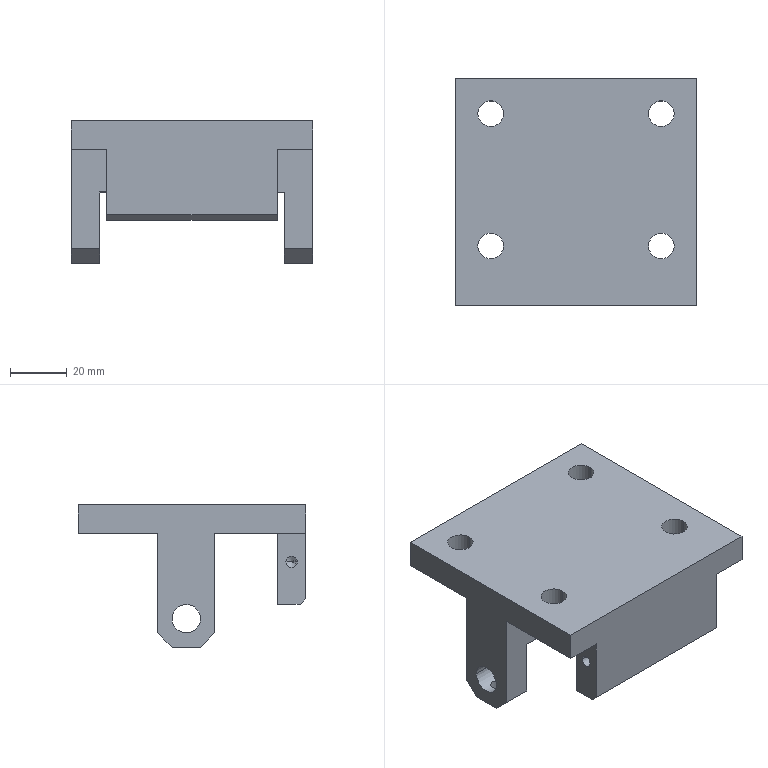Component | SolidWorks | LiftingPlateAssembly-1_LiftingPlateBracket-1 | 1 solid | 47 faces | box 85 x 80 x 50 mm | volume 113372 mm3 | plane 23 | cylinder 20 | cone 4 | commonest cylinder face diameters 4 x8 9 x8 10 x4 | material Plain Carbon Steel
build123d program:
from build123d import *

# Parameters (mm, degrees)
BOSS_EXTRUDE1_DEPTH          = 42.5
BOSS_EXTRUDE1_DEPTH_BACK     = 42.5
SKETCH2_R                    = 5
CUT_EXTRUDE1_DEPTH           = 103.903
CHAMFER1_SIZE                = 5
SKETCH3_W                    = 65
SKETCH3_H                    = 29.478
CUT_EXTRUDE2_DEPTH           = 20
CHAMFER2_SIZE                = 2
F_9_0_9_DIAMETER_HOLE1_D     = 9
F_9_0_9_DIAMETER_HOLE1_DEPTH = 333
F_9_0_9_DIAMETER_HOLE1_TIP   = 2.704
M4_TAPPED_HOLE1_D            = 4
M4_TAPPED_HOLE1_DEPTH        = 10.1
M4_TAPPED_HOLE1_TIP          = 1.202
SKETCH8_W                    = 21.784
SKETCH8_H                    = 26.093
SKETCH8_W_2                  = 22.483
SKETCH8_H_2                  = 25.531
CUT_EXTRUDE3_DEPTH           = 10
M4_TAPPED_HOLE4_D            = 4
M4_TAPPED_HOLE4_DEPTH        = 10.1
M4_TAPPED_HOLE4_TIP          = 1.202
M4_TAPPED_HOLE5_D            = 4
M4_TAPPED_HOLE5_DEPTH        = 10.1
M4_TAPPED_HOLE5_TIP          = 1.202


with BuildPart() as part:
    # Sketch1 → Boss-Extrude1 (new, two sides: drawn at the far end of the back side and taken through both)
    with BuildSketch(Plane.XY.offset(-BOSS_EXTRUDE1_DEPTH_BACK)):
        Polygon((-32, -5), (-32, -30), (-10, -30), (-10, 10), (10, 10), (10, -30), (38, -30), (38, -40), (-42, -40), (-42, -5), align=None)
    extrude(amount=BOSS_EXTRUDE1_DEPTH + BOSS_EXTRUDE1_DEPTH_BACK)

    # Sketch2 → Cut-Extrude1 (cut, through all)
    with BuildSketch(Plane.XY.offset(42.5)):
        Circle(SKETCH2_R)
    extrude(amount=-CUT_EXTRUDE1_DEPTH, mode=Mode.SUBTRACT)

    # Chamfer1
    chamfer1_edges = [part.edges().sort_by_distance(p)[0] for p in [
        (-10, 10, 0),
        (10, 10, 0),
    ]]
    chamfer(chamfer1_edges, length=CHAMFER1_SIZE)

    # Sketch3 → Cut-Extrude2 (cut)
    with BuildSketch(Plane(origin=(10, 0, 0), x_dir=(0, 0, -1), z_dir=(1, 0, 0))):
        with Locations((0, -0.2611)):
            Rectangle(SKETCH3_W, SKETCH3_H)
    extrude(amount=-CUT_EXTRUDE2_DEPTH, mode=Mode.SUBTRACT)

    # Chamfer2
    chamfer2_edges = [part.edges().sort_by_distance(p)[0] for p in [
        (-42, -5, 0),
    ]]
    chamfer(chamfer2_edges, length=CHAMFER2_SIZE)

    # 9.0 _9_ Diameter Hole1
    with Locations(Plane(origin=(0, -30, 0), x_dir=(1, 0, 0), z_dir=(0, 1, 0))):
        with Locations((-21, 30), (-21, -30), (25.5, 30), (25.5, -30)):
            Hole(F_9_0_9_DIAMETER_HOLE1_D / 2, depth=F_9_0_9_DIAMETER_HOLE1_DEPTH)
            with Locations((0, 0, -(F_9_0_9_DIAMETER_HOLE1_DEPTH + F_9_0_9_DIAMETER_HOLE1_TIP / 2))):  # 118° drill point
                Cone(0, F_9_0_9_DIAMETER_HOLE1_D / 2, F_9_0_9_DIAMETER_HOLE1_TIP, mode=Mode.SUBTRACT)

    # M4 Tapped Hole1
    with Locations(Plane(origin=(0, 10, 0), x_dir=(1, 0, 0), z_dir=(0, 1, 0))):
        with Locations((0, 37.5), (0, -37.5)):
            Hole(M4_TAPPED_HOLE1_D / 2, depth=M4_TAPPED_HOLE1_DEPTH)
            with Locations((0, 0, -(M4_TAPPED_HOLE1_DEPTH + M4_TAPPED_HOLE1_TIP / 2))):  # 118° drill point
                Cone(0, M4_TAPPED_HOLE1_D / 2, M4_TAPPED_HOLE1_TIP, mode=Mode.SUBTRACT)

    # Sketch8 → Cut-Extrude3 (cut)
    with BuildSketch(Plane.ZY.offset(42)):
        with Locations((40.892, -16.954)):
            Rectangle(SKETCH8_W, SKETCH8_H)
        with Locations((-41.241, -17.235)):
            Rectangle(SKETCH8_W_2, SKETCH8_H_2)
    extrude(amount=-CUT_EXTRUDE3_DEPTH, mode=Mode.SUBTRACT)

    # M4 Tapped Hole4
    with Locations(Plane(origin=(0, 0, -30), x_dir=(-1, 0, 0), z_dir=(0, 0, -1))):
        with Locations((37, -20)):
            Hole(M4_TAPPED_HOLE4_D / 2, depth=M4_TAPPED_HOLE4_DEPTH)
            with Locations((0, 0, -(M4_TAPPED_HOLE4_DEPTH + M4_TAPPED_HOLE4_TIP / 2))):  # 118° drill point
                Cone(0, M4_TAPPED_HOLE4_D / 2, M4_TAPPED_HOLE4_TIP, mode=Mode.SUBTRACT)

    # M4 Tapped Hole5
    with Locations(Plane.XY.offset(30)):
        with Locations((-37, -20)):
            Hole(M4_TAPPED_HOLE5_D / 2, depth=M4_TAPPED_HOLE5_DEPTH)
            with Locations((0, 0, -(M4_TAPPED_HOLE5_DEPTH + M4_TAPPED_HOLE5_TIP / 2))):  # 118° drill point
                Cone(0, M4_TAPPED_HOLE5_D / 2, M4_TAPPED_HOLE5_TIP, mode=Mode.SUBTRACT)


solid = part.part

# Placed as in the assembly
solid = solid.moved(Location((-250, 2, -65), (-90, -90, 0)))